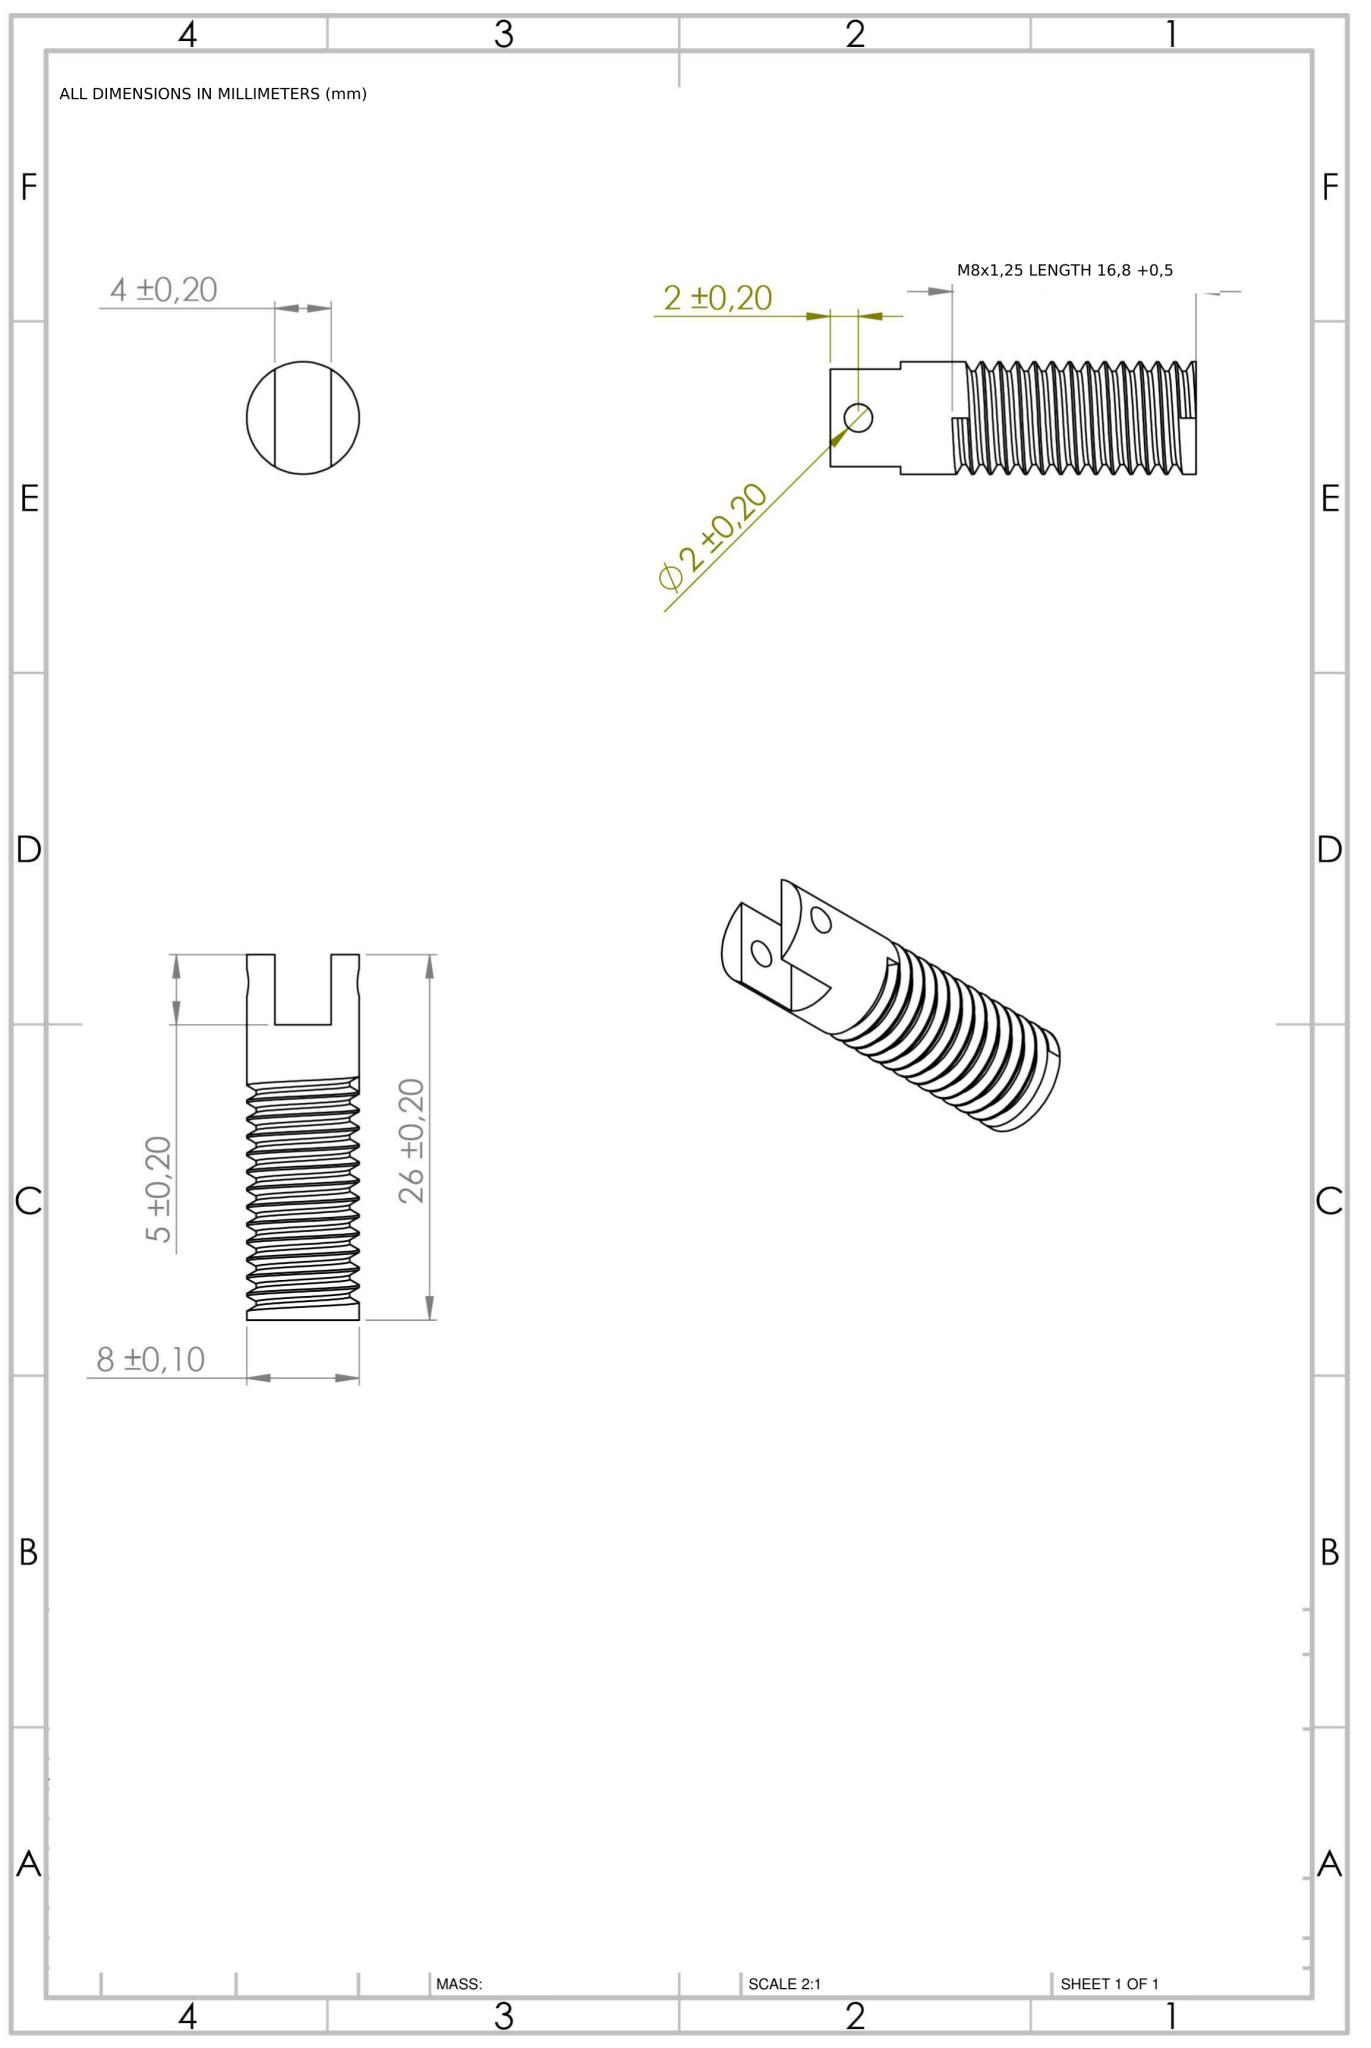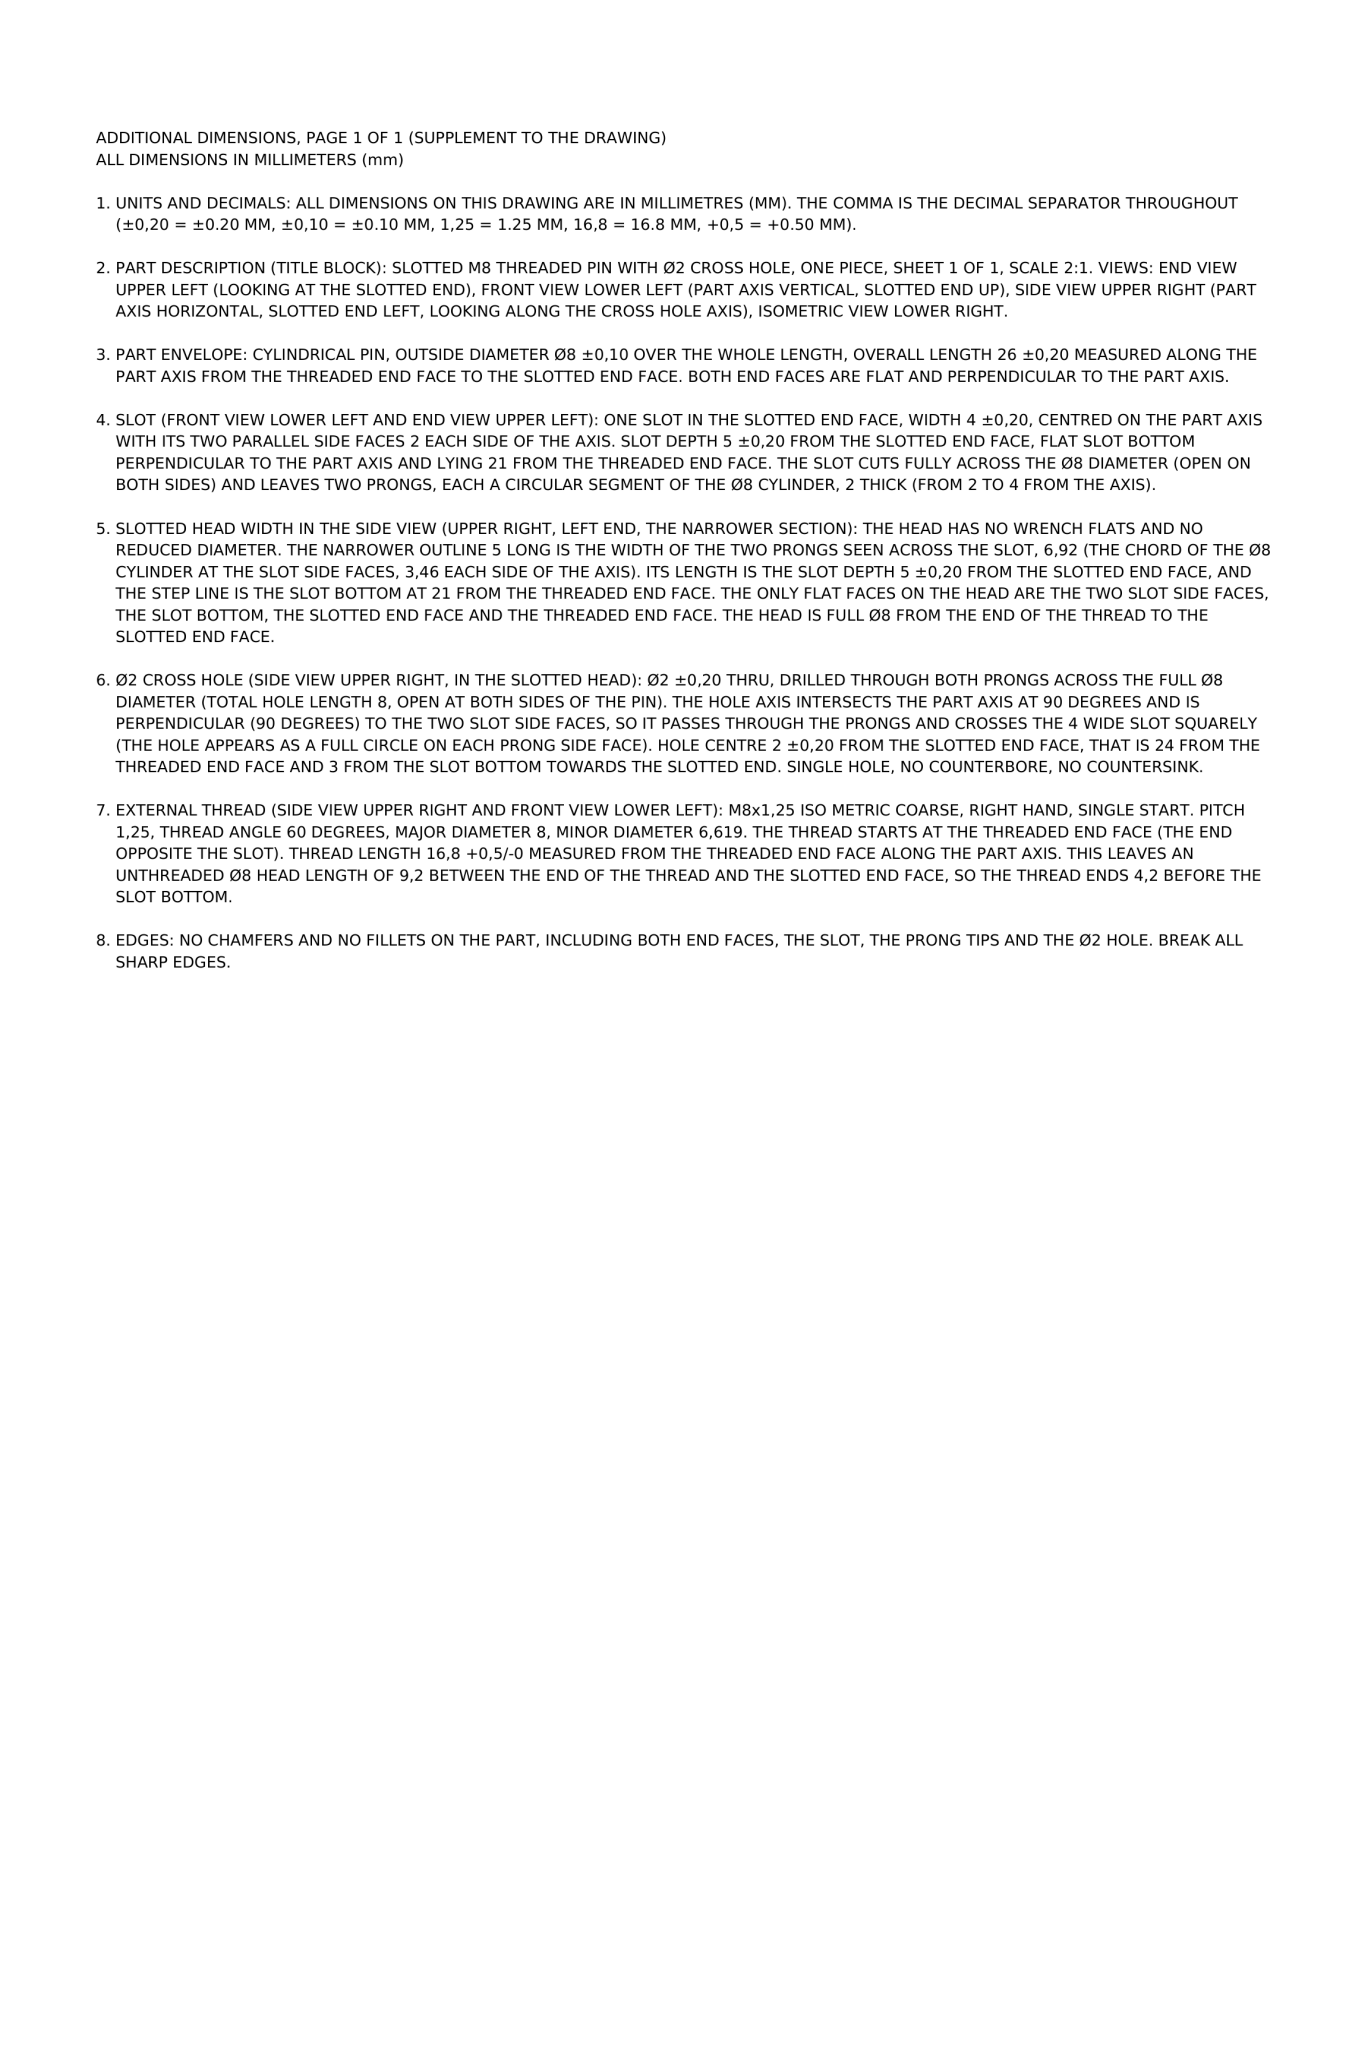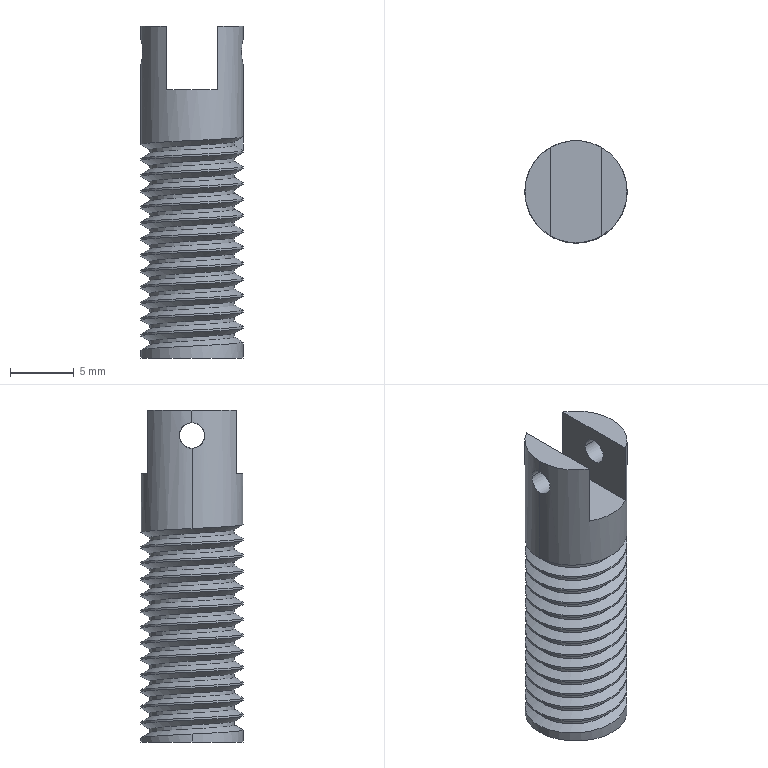Part | NX | mm | 1 solid | 43 faces | box 8 x 8 x 26 mm | volume 995 mm3 | cylinder 32 | plane 8 | spline 3 | commonest cylinder face diameters 8 x28 2 x4